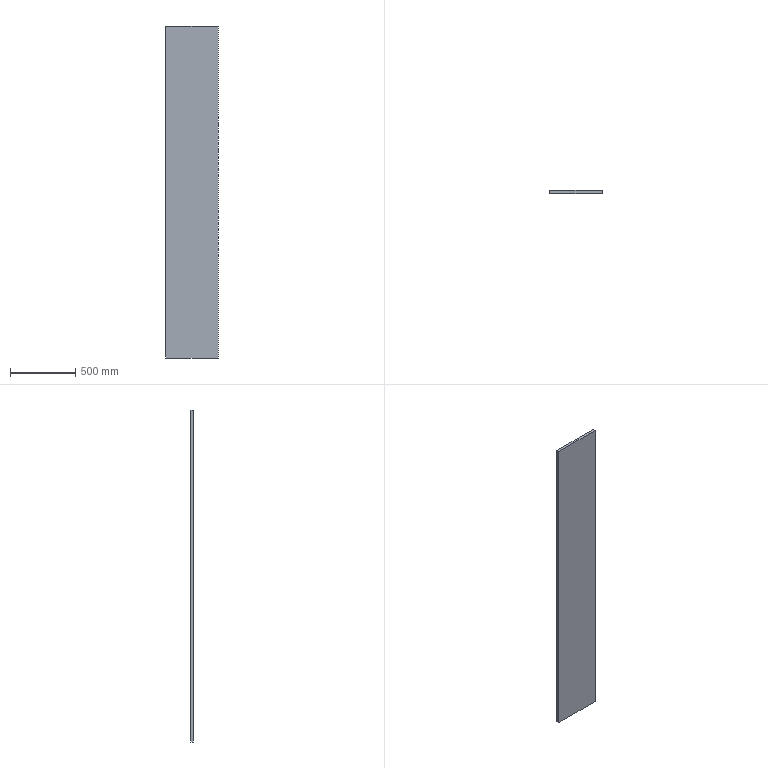Component | SolidWorks | ST60-05-1 | 1 solid | 6 faces | box 400 x 20 x 2540 mm | volume 20320000 mm3 | plane 6
build123d program:
from build123d import *

# Parameters (mm, degrees)
SKETCH1_W           = 2540
SKETCH1_H           = 400
BOSS_EXTRUDE1_DEPTH = 20


with BuildPart() as part:
    # Sketch1 → Boss-Extrude1 (new body)
    with BuildSketch(Plane.XY):
        with Locations((-254.489, 516.975)):
            Rectangle(SKETCH1_W, SKETCH1_H)
    extrude(amount=BOSS_EXTRUDE1_DEPTH)


solid = part.part

# Placed as in the assembly
solid = solid.moved(Location((969.968, 55.454, -955.511), (90, 0, 90)))
STEP:
#1=COLOUR_RGB('',0.7922,0.8196,0.9333);
#2=FILL_AREA_STYLE_COLOUR('',#1);
#3=FILL_AREA_STYLE('',(#2));
#4=SURFACE_STYLE_FILL_AREA(#3);
#5=SURFACE_SIDE_STYLE('',(#4));
#6=SURFACE_STYLE_USAGE(.BOTH.,#5);
#7=PRESENTATION_STYLE_ASSIGNMENT((#6));
#8=CARTESIAN_POINT('',(9.96,2.183,-97.638));
#9=VERTEX_POINT('',#8);
#10=CARTESIAN_POINT('',(25.708,2.183,-97.638));
#11=VERTEX_POINT('',#10);
#12=CARTESIAN_POINT('',(9.96,2.183,-97.638));
#13=DIRECTION('',(1.,0.,0.));
#14=VECTOR('',#13,39.37);
#15=LINE('',#12,#14);
#16=EDGE_CURVE('',#9,#11,#15,.T.);
#17=ORIENTED_EDGE('',*,*,#16,.T.);
#18=CARTESIAN_POINT('',(25.708,1.396,-97.638));
#19=VERTEX_POINT('',#18);
#20=CARTESIAN_POINT('',(25.708,1.396,-97.638));
#21=DIRECTION('',(0.,1.,0.));
#22=VECTOR('',#21,39.37);
#23=LINE('',#20,#22);
#24=EDGE_CURVE('',#19,#11,#23,.T.);
#25=ORIENTED_EDGE('',*,*,#24,.F.);
#26=CARTESIAN_POINT('',(9.96,1.396,-97.638));
#27=VERTEX_POINT('',#26);
#28=CARTESIAN_POINT('',(9.96,1.396,-97.638));
#29=DIRECTION('',(1.,0.,0.));
#30=VECTOR('',#29,39.37);
#31=LINE('',#28,#30);
#32=EDGE_CURVE('',#27,#19,#31,.T.);
#33=ORIENTED_EDGE('',*,*,#32,.F.);
#34=CARTESIAN_POINT('',(9.96,1.396,-97.638));
#35=DIRECTION('',(0.,1.,0.));
#36=VECTOR('',#35,39.37);
#37=LINE('',#34,#36);
#38=EDGE_CURVE('',#27,#9,#37,.T.);
#39=ORIENTED_EDGE('',*,*,#38,.T.);
#40=EDGE_LOOP('',(#17,#25,#33,#39));
#41=FACE_OUTER_BOUND('',#40,.T.);
#42=CARTESIAN_POINT('',(9.96,1.396,-97.638));
#43=DIRECTION('',(-0.,0.,1.));
#44=DIRECTION('',(-1.,0.,-0.));
#45=AXIS2_PLACEMENT_3D('',#42,#43,#44);
#46=PLANE('',#45);
#47=ADVANCED_FACE('',(#41),#46,.F.);
#48=CARTESIAN_POINT('',(25.708,2.183,2.362));
#49=VERTEX_POINT('',#48);
#50=CARTESIAN_POINT('',(25.708,2.183,-97.638));
#51=DIRECTION('',(0.,0.,1.));
#52=VECTOR('',#51,39.37);
#53=LINE('',#50,#52);
#54=EDGE_CURVE('',#11,#49,#53,.T.);
#55=ORIENTED_EDGE('',*,*,#54,.T.);
#56=CARTESIAN_POINT('',(25.708,1.396,2.362));
#57=VERTEX_POINT('',#56);
#58=CARTESIAN_POINT('',(25.708,1.396,2.362));
#59=DIRECTION('',(0.,1.,0.));
#60=VECTOR('',#59,39.37);
#61=LINE('',#58,#60);
#62=EDGE_CURVE('',#57,#49,#61,.T.);
#63=ORIENTED_EDGE('',*,*,#62,.F.);
#64=CARTESIAN_POINT('',(25.708,1.396,-97.638));
#65=DIRECTION('',(0.,0.,1.));
#66=VECTOR('',#65,39.37);
#67=LINE('',#64,#66);
#68=EDGE_CURVE('',#19,#57,#67,.T.);
#69=ORIENTED_EDGE('',*,*,#68,.F.);
#70=ORIENTED_EDGE('',*,*,#24,.T.);
#71=EDGE_LOOP('',(#55,#63,#69,#70));
#72=FACE_OUTER_BOUND('',#71,.T.);
#73=CARTESIAN_POINT('',(25.708,1.396,-97.638));
#74=DIRECTION('',(-1.,0.,0.));
#75=DIRECTION('',(0.,-1.,0.));
#76=AXIS2_PLACEMENT_3D('',#73,#74,#75);
#77=PLANE('',#76);
#78=ADVANCED_FACE('',(#72),#77,.F.);
#79=CARTESIAN_POINT('',(9.96,2.183,2.362));
#80=VERTEX_POINT('',#79);
#81=CARTESIAN_POINT('',(9.96,2.183,2.362));
#82=DIRECTION('',(-1.,0.,-0.));
#83=VECTOR('',#82,39.37);
#84=LINE('',#81,#83);
#85=EDGE_CURVE('',#49,#80,#84,.T.);
#86=ORIENTED_EDGE('',*,*,#85,.T.);
#87=CARTESIAN_POINT('',(9.96,1.396,2.362));
#88=VERTEX_POINT('',#87);
#89=CARTESIAN_POINT('',(9.96,1.396,2.362));
#90=DIRECTION('',(0.,1.,0.));
#91=VECTOR('',#90,39.37);
#92=LINE('',#89,#91);
#93=EDGE_CURVE('',#88,#80,#92,.T.);
#94=ORIENTED_EDGE('',*,*,#93,.F.);
#95=CARTESIAN_POINT('',(9.96,1.396,2.362));
#96=DIRECTION('',(-1.,0.,-0.));
#97=VECTOR('',#96,39.37);
#98=LINE('',#95,#97);
#99=EDGE_CURVE('',#57,#88,#98,.T.);
#100=ORIENTED_EDGE('',*,*,#99,.F.);
#101=ORIENTED_EDGE('',*,*,#62,.T.);
#102=EDGE_LOOP('',(#86,#94,#100,#101));
#103=FACE_OUTER_BOUND('',#102,.T.);
#104=CARTESIAN_POINT('',(9.96,1.396,2.362));
#105=DIRECTION('',(0.,0.,-1.));
#106=DIRECTION('',(1.,0.,0.));
#107=AXIS2_PLACEMENT_3D('',#104,#105,#106);
#108=PLANE('',#107);
#109=ADVANCED_FACE('',(#103),#108,.F.);
#110=CARTESIAN_POINT('',(9.96,2.183,-97.638));
#111=DIRECTION('',(0.,0.,-1.));
#112=VECTOR('',#111,39.37);
#113=LINE('',#110,#112);
#114=EDGE_CURVE('',#80,#9,#113,.T.);
#115=ORIENTED_EDGE('',*,*,#114,.T.);
#116=ORIENTED_EDGE('',*,*,#38,.F.);
#117=CARTESIAN_POINT('',(9.96,1.396,-97.638));
#118=DIRECTION('',(0.,0.,-1.));
#119=VECTOR('',#118,39.37);
#120=LINE('',#117,#119);
#121=EDGE_CURVE('',#88,#27,#120,.T.);
#122=ORIENTED_EDGE('',*,*,#121,.F.);
#123=ORIENTED_EDGE('',*,*,#93,.T.);
#124=EDGE_LOOP('',(#115,#116,#122,#123));
#125=FACE_OUTER_BOUND('',#124,.T.);
#126=CARTESIAN_POINT('',(9.96,1.396,-97.638));
#127=DIRECTION('',(1.,0.,0.));
#128=DIRECTION('',(0.,1.,0.));
#129=AXIS2_PLACEMENT_3D('',#126,#127,#128);
#130=PLANE('',#129);
#131=ADVANCED_FACE('',(#125),#130,.F.);
#132=ORIENTED_EDGE('',*,*,#32,.T.);
#133=ORIENTED_EDGE('',*,*,#68,.T.);
#134=ORIENTED_EDGE('',*,*,#99,.T.);
#135=ORIENTED_EDGE('',*,*,#121,.T.);
#136=EDGE_LOOP('',(#132,#133,#134,#135));
#137=FACE_OUTER_BOUND('',#136,.T.);
#138=CARTESIAN_POINT('',(38.188,1.396,-37.619));
#139=DIRECTION('',(0.,-1.,0.));
#140=DIRECTION('',(0.,0.,1.));
#141=AXIS2_PLACEMENT_3D('',#138,#139,#140);
#142=PLANE('',#141);
#143=ADVANCED_FACE('',(#137),#142,.T.);
#144=ORIENTED_EDGE('',*,*,#16,.F.);
#145=ORIENTED_EDGE('',*,*,#114,.F.);
#146=ORIENTED_EDGE('',*,*,#85,.F.);
#147=ORIENTED_EDGE('',*,*,#54,.F.);
#148=EDGE_LOOP('',(#144,#145,#146,#147));
#149=FACE_OUTER_BOUND('',#148,.T.);
#150=CARTESIAN_POINT('',(38.188,2.183,-37.619));
#151=DIRECTION('',(0.,-1.,0.));
#152=DIRECTION('',(0.,0.,1.));
#153=AXIS2_PLACEMENT_3D('',#150,#151,#152);
#154=PLANE('',#153);
#155=ADVANCED_FACE('',(#149),#154,.F.);
#156=CLOSED_SHELL('',(#47,#78,#109,#131,#143,#155));
#157=MANIFOLD_SOLID_BREP('',#156);
#158=STYLED_ITEM('',(#7),#157);
#159=PRESENTATION_LAYER_ASSIGNMENT('','',(#158));
#160=(LENGTH_UNIT()NAMED_UNIT(*)SI_UNIT($,.METRE.));
#161=LENGTH_MEASURE_WITH_UNIT(LENGTH_MEASURE(0.0254),#160);
#162=DIMENSIONAL_EXPONENTS(1.,0.,0.,0.,0.,0.,0.);
#163=(CONVERSION_BASED_UNIT('',#161)LENGTH_UNIT()NAMED_UNIT(#162));
#164=UNCERTAINTY_MEASURE_WITH_UNIT(LENGTH_MEASURE(0.00001),#163,'','');
#165=(NAMED_UNIT(*)PLANE_ANGLE_UNIT()SI_UNIT($,.RADIAN.));
#166=(NAMED_UNIT(*)SI_UNIT($,.STERADIAN.)SOLID_ANGLE_UNIT());
#167=(GEOMETRIC_REPRESENTATION_CONTEXT(3)GLOBAL_UNCERTAINTY_ASSIGNED_CONTEXT((#164))GLOBAL_UNIT_ASSIGNED_CONTEXT((#163,#165,#166))REPRESENTATION_CONTEXT('',''));
#168=MECHANICAL_DESIGN_GEOMETRIC_PRESENTATION_REPRESENTATION('',(#158),#167);
#169=CARTESIAN_POINT('',(0.,0.,0.));
#170=DIRECTION('',(0.,0.,1.));
#171=DIRECTION('',(1.,0.,0.));
#172=AXIS2_PLACEMENT_3D('',#169,#170,#171);
#173=(LENGTH_UNIT()NAMED_UNIT(*)SI_UNIT($,.METRE.));
#174=LENGTH_MEASURE_WITH_UNIT(LENGTH_MEASURE(0.0254),#173);
#175=DIMENSIONAL_EXPONENTS(1.,0.,0.,0.,0.,0.,0.);
#176=(CONVERSION_BASED_UNIT('',#174)LENGTH_UNIT()NAMED_UNIT(#175));
#177=UNCERTAINTY_MEASURE_WITH_UNIT(LENGTH_MEASURE(0.00001),#176,'','');
#178=(NAMED_UNIT(*)PLANE_ANGLE_UNIT()SI_UNIT($,.RADIAN.));
#179=(NAMED_UNIT(*)SI_UNIT($,.STERADIAN.)SOLID_ANGLE_UNIT());
#180=(GEOMETRIC_REPRESENTATION_CONTEXT(3)GLOBAL_UNCERTAINTY_ASSIGNED_CONTEXT((#177))GLOBAL_UNIT_ASSIGNED_CONTEXT((#176,#178,#179))REPRESENTATION_CONTEXT('',''));
#181=ADVANCED_BREP_SHAPE_REPRESENTATION('',(#157,#172),#180);